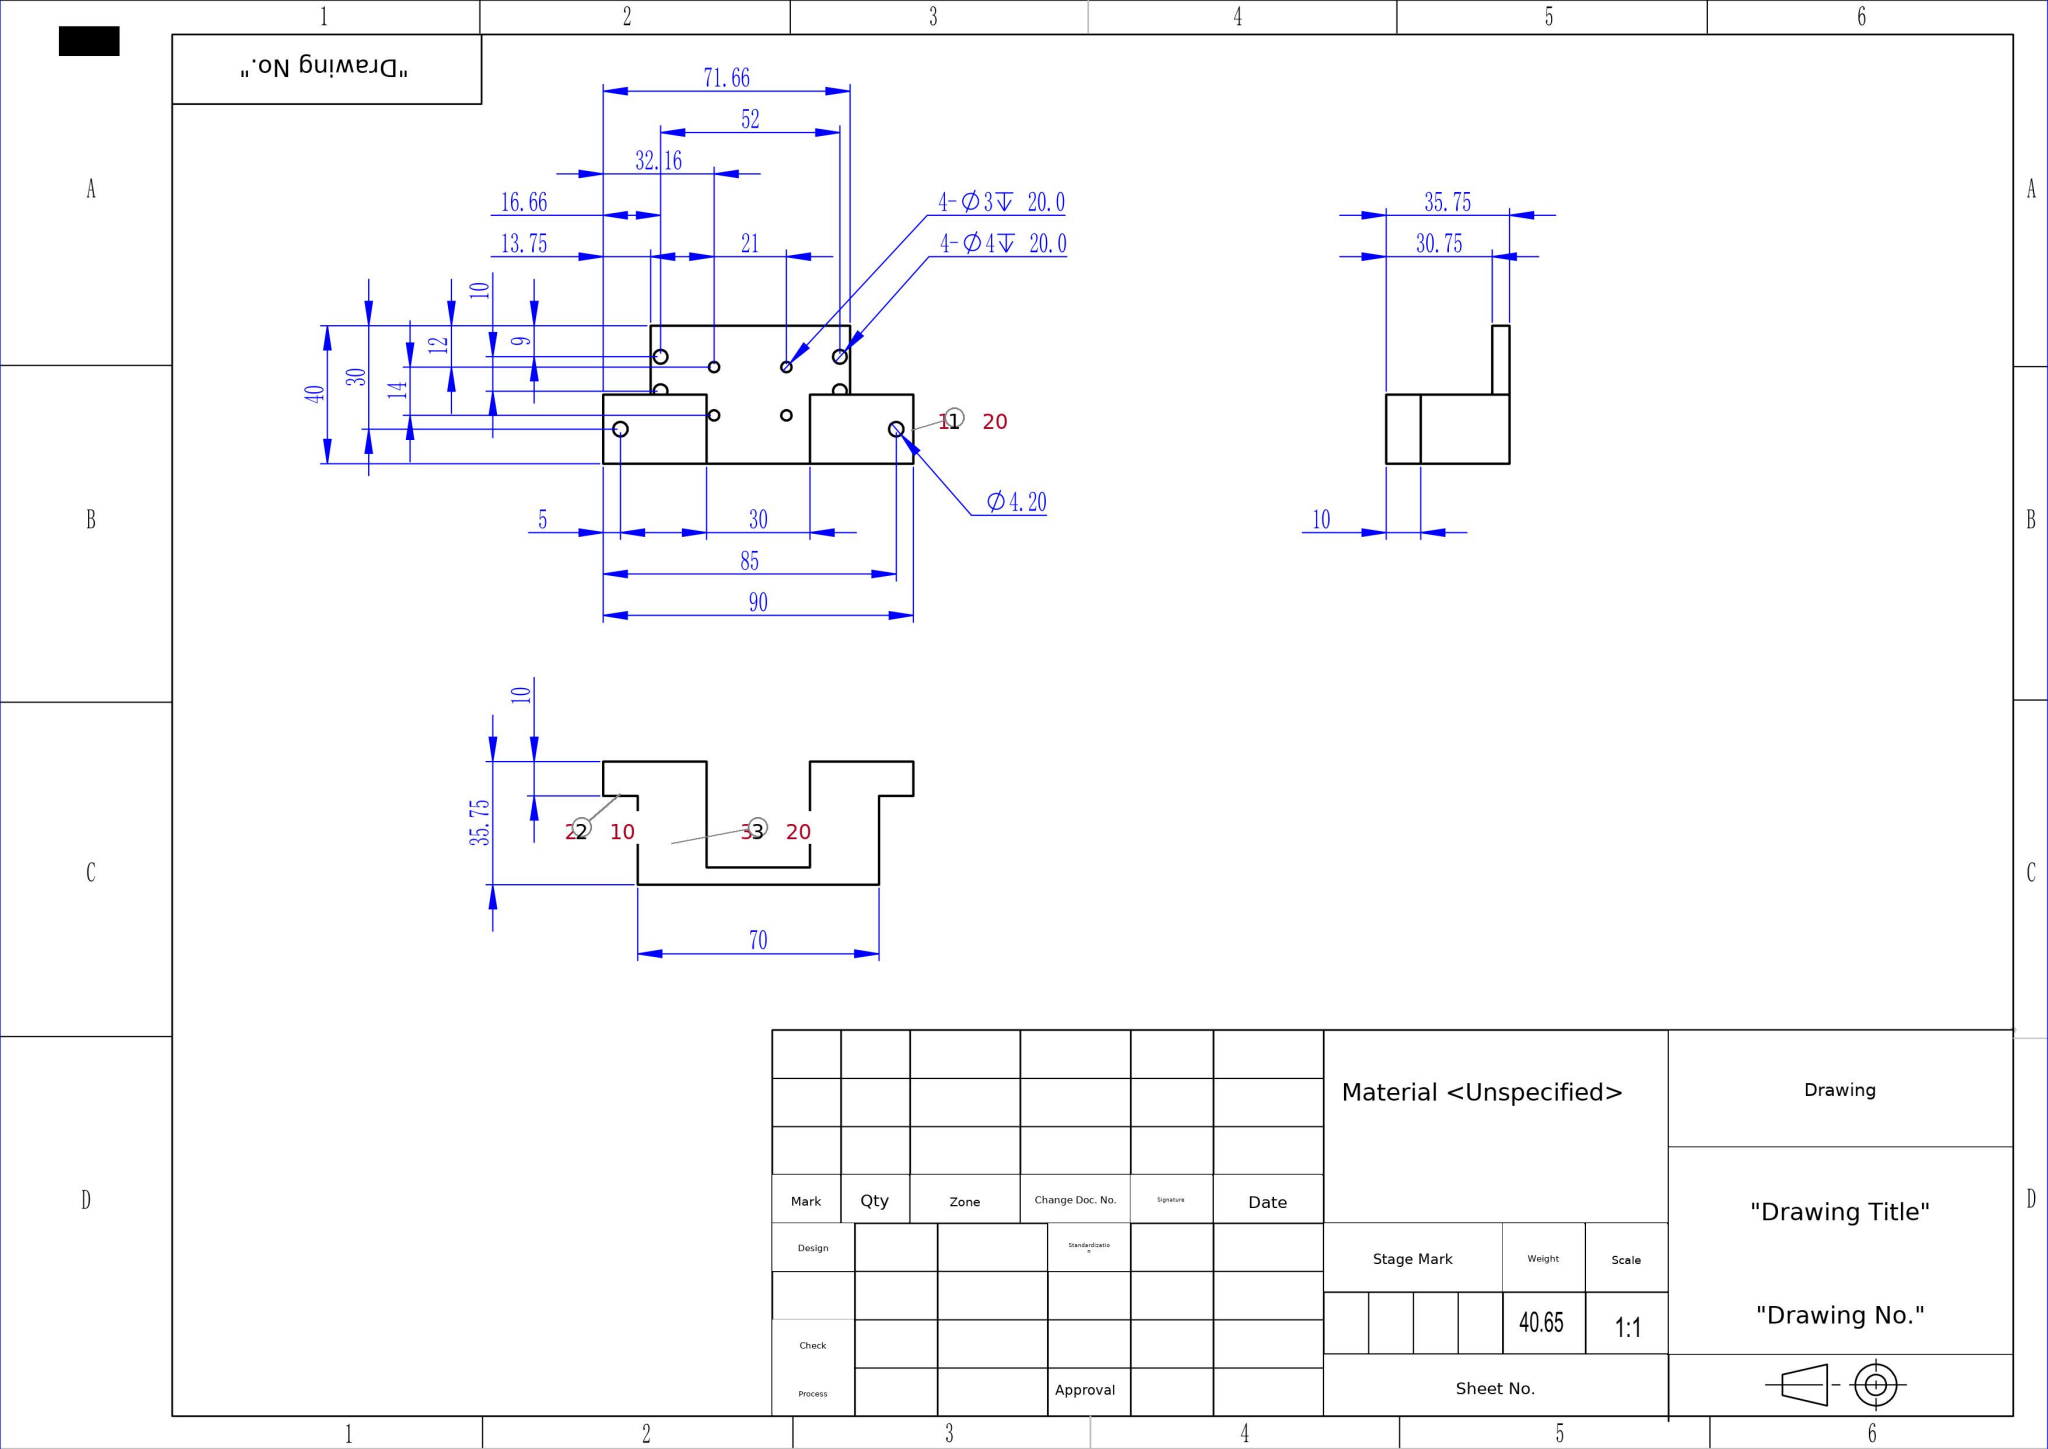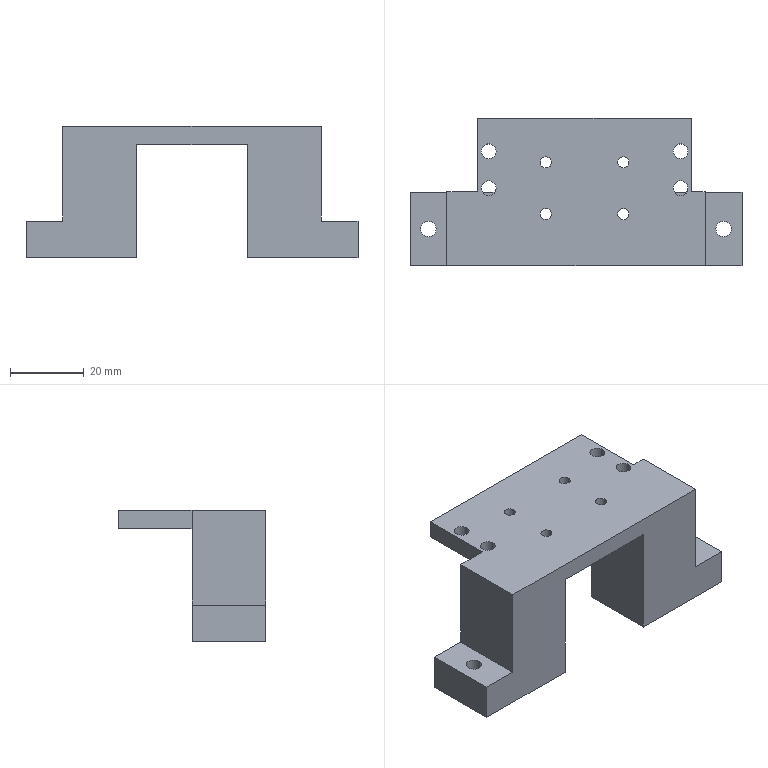Part | SolidWorks | mm | 1 solid | 40 faces | box 90 x 40 x 35.75 mm | volume 40648 mm3 | cylinder 20 | plane 20 | commonest cylinder face diameters 3 x8 4 x8 4.2 x4
build123d program:
from build123d import *

# Parameters (mm, degrees)
SKETCH1_W           = 30
SKETCH1_H           = 20
SKETCH1_R           = 2.1
BOSS_EXTRUDE1_DEPTH = 10
SKETCH2_W           = 20
SKETCH2_H           = 20
BOSS_EXTRUDE2_DEPTH = 25.75
SKETCH3_W           = 5
SKETCH3_H           = 20
BOSS_EXTRUDE3_DEPTH = 15
SKETCH4_W           = 57.914
SKETCH4_H           = 5
BOSS_EXTRUDE4_DEPTH = 20
SKETCH5_R           = 2
SKETCH5_R_2         = 1.5
CUT_EXTRUDE1_DEPTH  = 20


with BuildPart() as part:
    # Sketch1 → Boss-Extrude1 (new body)
    with BuildSketch(Plane.XY):
        Rectangle(SKETCH1_W, SKETCH1_H)
        with Locations((-10, 0)):
            Circle(SKETCH1_R, mode=Mode.SUBTRACT)
    extrude(amount=BOSS_EXTRUDE1_DEPTH)

    # Sketch2 → Boss-Extrude2 (add)
    with BuildSketch(Plane.XY.offset(10)):
        with Locations((5, 0)):
            Rectangle(SKETCH2_W, SKETCH2_H)
    extrude(amount=BOSS_EXTRUDE2_DEPTH)

    # Sketch3 → Boss-Extrude3 (add)
    with BuildSketch(Plane(origin=(15, 0, 0), x_dir=(0, 0, -1), z_dir=(1, 0, 0))):
        with Locations((-33.25, 0)):
            Rectangle(SKETCH3_W, SKETCH3_H)
    extrude(amount=BOSS_EXTRUDE3_DEPTH)

    # Mirror1: part across plane


with BuildPart() as part_1:
    add(part.part)
    add(part.part.mirror(Plane(origin=(30, 0, 0), x_dir=(0, 0, 1), z_dir=(1, 0, 0))))

    # Sketch4 → Boss-Extrude4 (add)
    with BuildSketch(Plane(origin=(0, 10, 0), x_dir=(1, 0, 0), z_dir=(0, 1, 0))):
        with Locations((32.297, -33.25)):
            Rectangle(SKETCH4_W, SKETCH4_H)
    extrude(amount=BOSS_EXTRUDE4_DEPTH)

    # Sketch5 → Cut-Extrude1 (cut)
    with BuildSketch(Plane.XY.offset(35.75)):
        with Locations((6.34, 21)):
            Circle(SKETCH5_R)
        with Locations((6.34, 11)):
            Circle(SKETCH5_R)
        with Locations((58.34, 11)):
            Circle(SKETCH5_R)
        with Locations((58.34, 21)):
            Circle(SKETCH5_R)
        with Locations((21.84, 4)):
            Circle(SKETCH5_R_2)
        with Locations((42.84, 4)):
            Circle(SKETCH5_R_2)
        with Locations((21.84, 18)):
            Circle(SKETCH5_R_2)
        with Locations((42.84, 18)):
            Circle(SKETCH5_R_2)
    extrude(amount=-CUT_EXTRUDE1_DEPTH, mode=Mode.SUBTRACT)


solid = part_1.part